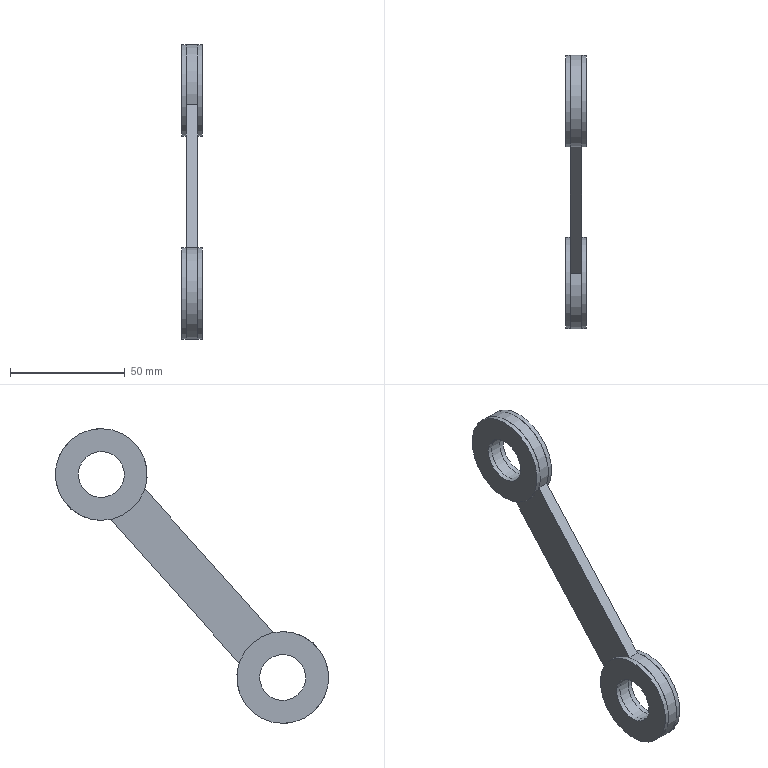Component | NX | MODEL2 | 5 solids | 24 faces | volume 25002 mm3 | cylinder 12 | plane 12 | commonest cylinder face diameters 40 x6 20 x6